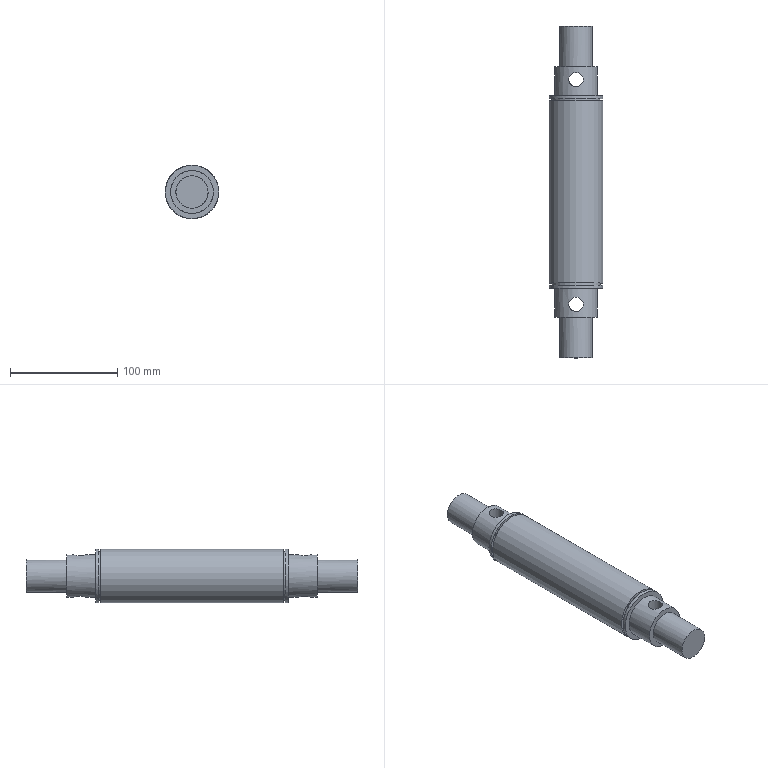Component | NX | SHAFT | 1 solid | 21 faces | volume 462946 mm3 | cylinder 11 | plane 10 | commonest cylinder face diameters 50 x3 40 x2 30.158 x2 45.5 x2 13.5 x2